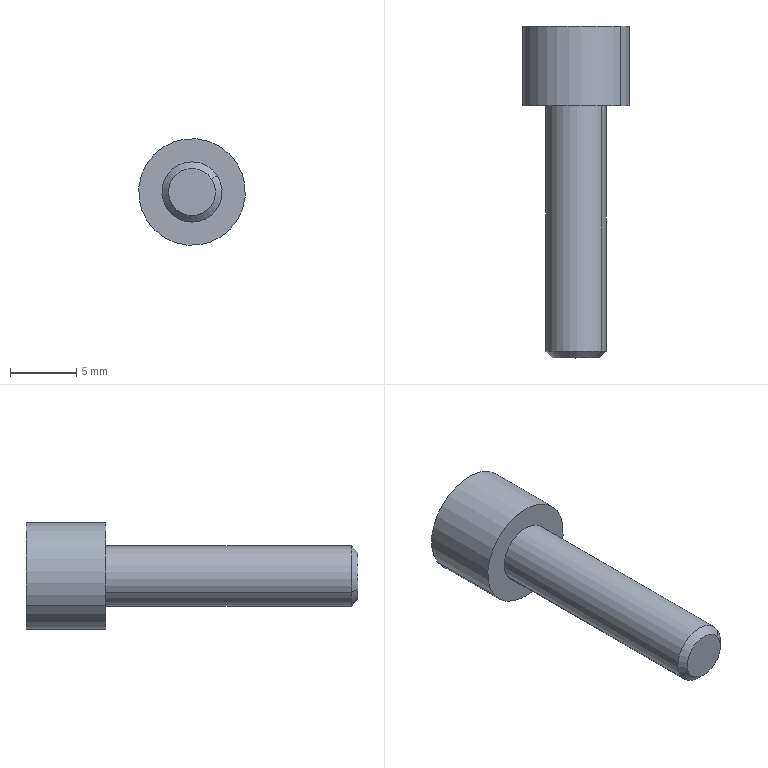Component | SolidWorks | CountersunkScrewM8x4-2 | 1 solid | 9 faces | box 8.03 x 25 x 8.03 mm | volume 610 mm3 | cylinder 4 | plane 3 | cone 2 | commonest cylinder face diameters 4.542 x2 8.034 x2
build123d program:
from build123d import *

# Parameters (mm, degrees)
SKETCH2_R           = 4.017
BOSS_EXTRUDE1_DEPTH = 10
SKETCH5_R           = 2.271
BOSS_EXTRUDE2_DEPTH = 29
CHAMFER1_SIZE       = 0.5
CUT_EXTRUDE1_DEPTH  = 4


with BuildPart() as part:
    # Sketch2 → Boss-Extrude1 (new body)
    with BuildSketch(Plane.XY.offset(20)):
        with Locations((20.473, -29.973)):
            Circle(SKETCH2_R)
    extrude(amount=-BOSS_EXTRUDE1_DEPTH)

    # Sketch5 → Boss-Extrude2 (add)
    with BuildSketch(Plane.XY.offset(20)):
        with Locations((20.473, -29.973)):
            Circle(SKETCH5_R)
    extrude(amount=-BOSS_EXTRUDE2_DEPTH)

    # Chamfer1
    chamfer1_edges = [part.edges().sort_by_distance(p)[0] for p in [
        (18.202, -29.973, -9),
    ]]
    chamfer(chamfer1_edges, length=CHAMFER1_SIZE)

    # Sketch6 → Cut-Extrude1 (cut)
    with BuildSketch(Plane.XY.offset(20)):
        Polygon((20.473, -8.425), (1.812, -19.199), (1.812, -40.747), (20.473, -51.521), (39.134, -40.747), (39.134, -19.199), align=None)
    extrude(amount=-CUT_EXTRUDE1_DEPTH, mode=Mode.SUBTRACT)


solid = part.part

# Placed as in the assembly
solid = solid.moved(Location((66.098, 96.74, -50.446), (-90, 0, 0)))
STEP:
#1=CARTESIAN_POINT('',(3.467,3.454,-0.7679));
#2=VERTEX_POINT('',#1);
#3=CARTESIAN_POINT('',(3.35,3.454,-0.8442));
#4=VERTEX_POINT('',#3);
#5=CARTESIAN_POINT('',(3.408,3.454,-0.806));
#6=DIRECTION('',(-0.,-1.,0.));
#7=DIRECTION('',(-0.8372,0.,-0.5469));
#8=AXIS2_PLACEMENT_3D('',#5,#6,#7);
#9=CIRCLE('',#8,0.06972);
#10=EDGE_CURVE('',#2,#4,#9,.T.);
#11=ORIENTED_EDGE('',*,*,#10,.F.);
#12=CARTESIAN_POINT('',(3.483,3.474,-0.7571));
#13=VERTEX_POINT('',#12);
#14=CARTESIAN_POINT('',(3.483,3.474,-0.7571));
#15=DIRECTION('',(0.592,0.7071,0.3867));
#16=VECTOR('',#15,39.37);
#17=LINE('',#14,#16);
#18=EDGE_CURVE('',#2,#13,#17,.T.);
#19=ORIENTED_EDGE('',*,*,#18,.T.);
#20=CARTESIAN_POINT('',(3.333,3.474,-0.8549));
#21=VERTEX_POINT('',#20);
#22=CARTESIAN_POINT('',(3.408,3.474,-0.806));
#23=DIRECTION('',(0.,1.,-0.));
#24=DIRECTION('',(-0.8372,0.,-0.5469));
#25=AXIS2_PLACEMENT_3D('',#22,#23,#24);
#26=CIRCLE('',#25,0.08941);
#27=EDGE_CURVE('',#21,#13,#26,.T.);
#28=ORIENTED_EDGE('',*,*,#27,.F.);
#29=CARTESIAN_POINT('',(3.333,3.474,-0.8549));
#30=DIRECTION('',(-0.592,0.7071,-0.3867));
#31=VECTOR('',#30,39.37);
#32=LINE('',#29,#31);
#33=EDGE_CURVE('',#4,#21,#32,.T.);
#34=ORIENTED_EDGE('',*,*,#33,.F.);
#35=EDGE_LOOP('',(#11,#19,#28,#34));
#36=FACE_OUTER_BOUND('',#35,.T.);
#37=CARTESIAN_POINT('',(3.408,3.474,-0.806));
#38=DIRECTION('',(0.,1.,-0.));
#39=DIRECTION('',(-0.8372,0.,-0.5469));
#40=AXIS2_PLACEMENT_3D('',#37,#38,#39);
#41=CONICAL_SURFACE('',#40,0.08941,0.7854);
#42=ADVANCED_FACE('',(#36),#41,.T.);
#43=ORIENTED_EDGE('',*,*,#27,.T.);
#44=CARTESIAN_POINT('',(3.483,4.202,-0.7571));
#45=VERTEX_POINT('',#44);
#46=CARTESIAN_POINT('',(3.483,3.454,-0.7571));
#47=DIRECTION('',(0.,1.,-0.));
#48=VECTOR('',#47,39.37);
#49=LINE('',#46,#48);
#50=EDGE_CURVE('',#13,#45,#49,.T.);
#51=ORIENTED_EDGE('',*,*,#50,.T.);
#52=CARTESIAN_POINT('',(3.333,4.202,-0.8549));
#53=VERTEX_POINT('',#52);
#54=CARTESIAN_POINT('',(3.408,4.202,-0.806));
#55=DIRECTION('',(-0.,1.,-0.));
#56=DIRECTION('',(-0.8372,0.,-0.5469));
#57=AXIS2_PLACEMENT_3D('',#54,#55,#56);
#58=CIRCLE('',#57,0.08941);
#59=EDGE_CURVE('',#53,#45,#58,.T.);
#60=ORIENTED_EDGE('',*,*,#59,.F.);
#61=CARTESIAN_POINT('',(3.333,3.454,-0.8549));
#62=DIRECTION('',(0.,1.,-0.));
#63=VECTOR('',#62,39.37);
#64=LINE('',#61,#63);
#65=EDGE_CURVE('',#21,#53,#64,.T.);
#66=ORIENTED_EDGE('',*,*,#65,.F.);
#67=EDGE_LOOP('',(#43,#51,#60,#66));
#68=FACE_OUTER_BOUND('',#67,.T.);
#69=CARTESIAN_POINT('',(3.408,3.454,-0.806));
#70=DIRECTION('',(0.,1.,-0.));
#71=DIRECTION('',(-0.8372,0.,-0.5469));
#72=AXIS2_PLACEMENT_3D('',#69,#70,#71);
#73=CYLINDRICAL_SURFACE('',#72,0.08941);
#74=ADVANCED_FACE('',(#68),#73,.T.);
#75=CARTESIAN_POINT('',(3.541,4.202,-0.7195));
#76=VERTEX_POINT('',#75);
#77=CARTESIAN_POINT('',(3.276,4.202,-0.8925));
#78=VERTEX_POINT('',#77);
#79=CARTESIAN_POINT('',(3.408,4.202,-0.806));
#80=DIRECTION('',(0.,-1.,0.));
#81=DIRECTION('',(-0.8372,-0.,-0.5469));
#82=AXIS2_PLACEMENT_3D('',#79,#80,#81);
#83=CIRCLE('',#82,0.1582);
#84=EDGE_CURVE('',#76,#78,#83,.T.);
#85=ORIENTED_EDGE('',*,*,#84,.F.);
#86=CARTESIAN_POINT('',(3.541,4.439,-0.7195));
#87=VERTEX_POINT('',#86);
#88=CARTESIAN_POINT('',(3.541,3.755,-0.7195));
#89=DIRECTION('',(0.,1.,-0.));
#90=VECTOR('',#89,39.37);
#91=LINE('',#88,#90);
#92=EDGE_CURVE('',#76,#87,#91,.T.);
#93=ORIENTED_EDGE('',*,*,#92,.T.);
#94=CARTESIAN_POINT('',(3.276,4.439,-0.8925));
#95=VERTEX_POINT('',#94);
#96=CARTESIAN_POINT('',(3.408,4.439,-0.806));
#97=DIRECTION('',(-0.,-1.,0.));
#98=DIRECTION('',(-0.8372,0.,-0.5469));
#99=AXIS2_PLACEMENT_3D('',#96,#97,#98);
#100=CIRCLE('',#99,0.1582);
#101=EDGE_CURVE('',#87,#95,#100,.T.);
#102=ORIENTED_EDGE('',*,*,#101,.T.);
#103=CARTESIAN_POINT('',(3.276,3.755,-0.8925));
#104=DIRECTION('',(0.,1.,-0.));
#105=VECTOR('',#104,39.37);
#106=LINE('',#103,#105);
#107=EDGE_CURVE('',#78,#95,#106,.T.);
#108=ORIENTED_EDGE('',*,*,#107,.F.);
#109=EDGE_LOOP('',(#85,#93,#102,#108));
#110=FACE_OUTER_BOUND('',#109,.T.);
#111=CARTESIAN_POINT('',(3.408,3.755,-0.806));
#112=DIRECTION('',(0.,1.,-0.));
#113=DIRECTION('',(-0.8372,0.,-0.5469));
#114=AXIS2_PLACEMENT_3D('',#111,#112,#113);
#115=CYLINDRICAL_SURFACE('',#114,0.1582);
#116=ADVANCED_FACE('',(#110),#115,.T.);
#117=ORIENTED_EDGE('',*,*,#92,.F.);
#118=CARTESIAN_POINT('',(3.408,4.202,-0.806));
#119=DIRECTION('',(0.,-1.,0.));
#120=DIRECTION('',(-0.8372,-0.,-0.5469));
#121=AXIS2_PLACEMENT_3D('',#118,#119,#120);
#122=CIRCLE('',#121,0.1582);
#123=EDGE_CURVE('',#78,#76,#122,.T.);
#124=ORIENTED_EDGE('',*,*,#123,.F.);
#125=ORIENTED_EDGE('',*,*,#107,.T.);
#126=CARTESIAN_POINT('',(3.408,4.439,-0.806));
#127=DIRECTION('',(-0.,-1.,0.));
#128=DIRECTION('',(-0.8372,0.,-0.5469));
#129=AXIS2_PLACEMENT_3D('',#126,#127,#128);
#130=CIRCLE('',#129,0.1582);
#131=EDGE_CURVE('',#95,#87,#130,.T.);
#132=ORIENTED_EDGE('',*,*,#131,.T.);
#133=EDGE_LOOP('',(#117,#124,#125,#132));
#134=FACE_OUTER_BOUND('',#133,.T.);
#135=CARTESIAN_POINT('',(3.408,3.755,-0.806));
#136=DIRECTION('',(0.,1.,-0.));
#137=DIRECTION('',(-0.8372,0.,-0.5469));
#138=AXIS2_PLACEMENT_3D('',#135,#136,#137);
#139=CYLINDRICAL_SURFACE('',#138,0.1582);
#140=ADVANCED_FACE('',(#134),#139,.T.);
#141=ORIENTED_EDGE('',*,*,#59,.T.);
#142=CARTESIAN_POINT('',(3.408,4.202,-0.806));
#143=DIRECTION('',(-0.,1.,-0.));
#144=DIRECTION('',(-0.8372,0.,-0.5469));
#145=AXIS2_PLACEMENT_3D('',#142,#143,#144);
#146=CIRCLE('',#145,0.08941);
#147=EDGE_CURVE('',#45,#53,#146,.T.);
#148=ORIENTED_EDGE('',*,*,#147,.T.);
#149=EDGE_LOOP('',(#141,#148));
#150=FACE_BOUND('',#149,.T.);
#151=ORIENTED_EDGE('',*,*,#123,.T.);
#152=ORIENTED_EDGE('',*,*,#84,.T.);
#153=EDGE_LOOP('',(#151,#152));
#154=FACE_OUTER_BOUND('',#153,.T.);
#155=CARTESIAN_POINT('',(3.408,4.202,-0.806));
#156=DIRECTION('',(-0.,1.,-0.));
#157=DIRECTION('',(0.5469,-0.,-0.8372));
#158=AXIS2_PLACEMENT_3D('',#155,#156,#157);
#159=PLANE('',#158);
#160=ADVANCED_FACE('',(#150,#154),#159,.F.);
#161=ORIENTED_EDGE('',*,*,#50,.F.);
#162=CARTESIAN_POINT('',(3.408,3.474,-0.806));
#163=DIRECTION('',(0.,1.,-0.));
#164=DIRECTION('',(-0.8372,0.,-0.5469));
#165=AXIS2_PLACEMENT_3D('',#162,#163,#164);
#166=CIRCLE('',#165,0.08941);
#167=EDGE_CURVE('',#13,#21,#166,.T.);
#168=ORIENTED_EDGE('',*,*,#167,.T.);
#169=ORIENTED_EDGE('',*,*,#65,.T.);
#170=ORIENTED_EDGE('',*,*,#147,.F.);
#171=EDGE_LOOP('',(#161,#168,#169,#170));
#172=FACE_OUTER_BOUND('',#171,.T.);
#173=CARTESIAN_POINT('',(3.408,3.454,-0.806));
#174=DIRECTION('',(0.,1.,-0.));
#175=DIRECTION('',(-0.8372,0.,-0.5469));
#176=AXIS2_PLACEMENT_3D('',#173,#174,#175);
#177=CYLINDRICAL_SURFACE('',#176,0.08941);
#178=ADVANCED_FACE('',(#172),#177,.T.);
#179=CARTESIAN_POINT('',(3.408,3.454,-0.806));
#180=DIRECTION('',(-0.,-1.,0.));
#181=DIRECTION('',(-0.8372,0.,-0.5469));
#182=AXIS2_PLACEMENT_3D('',#179,#180,#181);
#183=CIRCLE('',#182,0.06972);
#184=EDGE_CURVE('',#4,#2,#183,.T.);
#185=ORIENTED_EDGE('',*,*,#184,.T.);
#186=ORIENTED_EDGE('',*,*,#10,.T.);
#187=EDGE_LOOP('',(#185,#186));
#188=FACE_OUTER_BOUND('',#187,.T.);
#189=CARTESIAN_POINT('',(3.408,3.454,-0.806));
#190=DIRECTION('',(0.,1.,-0.));
#191=DIRECTION('',(-0.8372,0.,-0.5469));
#192=AXIS2_PLACEMENT_3D('',#189,#190,#191);
#193=PLANE('',#192);
#194=ADVANCED_FACE('',(#188),#193,.F.);
#195=ORIENTED_EDGE('',*,*,#18,.F.);
#196=ORIENTED_EDGE('',*,*,#184,.F.);
#197=ORIENTED_EDGE('',*,*,#33,.T.);
#198=ORIENTED_EDGE('',*,*,#167,.F.);
#199=EDGE_LOOP('',(#195,#196,#197,#198));
#200=FACE_OUTER_BOUND('',#199,.T.);
#201=CARTESIAN_POINT('',(3.408,3.474,-0.806));
#202=DIRECTION('',(0.,1.,-0.));
#203=DIRECTION('',(-0.8372,0.,-0.5469));
#204=AXIS2_PLACEMENT_3D('',#201,#202,#203);
#205=CONICAL_SURFACE('',#204,0.08941,0.7854);
#206=ADVANCED_FACE('',(#200),#205,.T.);
#207=ORIENTED_EDGE('',*,*,#131,.F.);
#208=ORIENTED_EDGE('',*,*,#101,.F.);
#209=EDGE_LOOP('',(#207,#208));
#210=FACE_OUTER_BOUND('',#209,.T.);
#211=CARTESIAN_POINT('',(3.438,4.439,0.6227));
#212=DIRECTION('',(0.,1.,-0.));
#213=DIRECTION('',(-0.8372,0.,-0.5469));
#214=AXIS2_PLACEMENT_3D('',#211,#212,#213);
#215=PLANE('',#214);
#216=ADVANCED_FACE('',(#210),#215,.T.);
#217=CLOSED_SHELL('',(#42,#74,#116,#140,#160,#178,#194,#206,#216));
#218=MANIFOLD_SOLID_BREP('',#217);
#219=CARTESIAN_POINT('',(0.,0.,0.));
#220=DIRECTION('',(0.,0.,1.));
#221=DIRECTION('',(1.,0.,0.));
#222=AXIS2_PLACEMENT_3D('',#219,#220,#221);
#223=(LENGTH_UNIT()NAMED_UNIT(*)SI_UNIT($,.METRE.));
#224=LENGTH_MEASURE_WITH_UNIT(LENGTH_MEASURE(0.0254),#223);
#225=DIMENSIONAL_EXPONENTS(1.,0.,0.,0.,0.,0.,0.);
#226=(CONVERSION_BASED_UNIT('',#224)LENGTH_UNIT()NAMED_UNIT(#225));
#227=UNCERTAINTY_MEASURE_WITH_UNIT(LENGTH_MEASURE(0.00001),#226,'','');
#228=(NAMED_UNIT(*)PLANE_ANGLE_UNIT()SI_UNIT($,.RADIAN.));
#229=(NAMED_UNIT(*)SI_UNIT($,.STERADIAN.)SOLID_ANGLE_UNIT());
#230=(GEOMETRIC_REPRESENTATION_CONTEXT(3)GLOBAL_UNCERTAINTY_ASSIGNED_CONTEXT((#227))GLOBAL_UNIT_ASSIGNED_CONTEXT((#226,#228,#229))REPRESENTATION_CONTEXT('',''));
#231=ADVANCED_BREP_SHAPE_REPRESENTATION('',(#218,#222),#230);
#232=COLOUR_RGB('',0.7922,0.8196,0.9333);
#233=FILL_AREA_STYLE_COLOUR('',#232);
#234=FILL_AREA_STYLE('',(#233));
#235=SURFACE_STYLE_FILL_AREA(#234);
#236=SURFACE_SIDE_STYLE('',(#235));
#237=SURFACE_STYLE_USAGE(.BOTH.,#236);
#238=PRESENTATION_STYLE_ASSIGNMENT((#237));
#239=STYLED_ITEM('',(#238),#218);
#240=(LENGTH_UNIT()NAMED_UNIT(*)SI_UNIT($,.METRE.));
#241=LENGTH_MEASURE_WITH_UNIT(LENGTH_MEASURE(0.0254),#240);
#242=DIMENSIONAL_EXPONENTS(1.,0.,0.,0.,0.,0.,0.);
#243=(CONVERSION_BASED_UNIT('',#241)LENGTH_UNIT()NAMED_UNIT(#242));
#244=UNCERTAINTY_MEASURE_WITH_UNIT(LENGTH_MEASURE(0.00001),#243,'','');
#245=(NAMED_UNIT(*)PLANE_ANGLE_UNIT()SI_UNIT($,.RADIAN.));
#246=(NAMED_UNIT(*)SI_UNIT($,.STERADIAN.)SOLID_ANGLE_UNIT());
#247=(GEOMETRIC_REPRESENTATION_CONTEXT(3)GLOBAL_UNCERTAINTY_ASSIGNED_CONTEXT((#244))GLOBAL_UNIT_ASSIGNED_CONTEXT((#243,#245,#246))REPRESENTATION_CONTEXT('',''));
#248=MECHANICAL_DESIGN_GEOMETRIC_PRESENTATION_REPRESENTATION('',(#239),#247);
#249=PRESENTATION_LAYER_ASSIGNMENT('','',(#239));